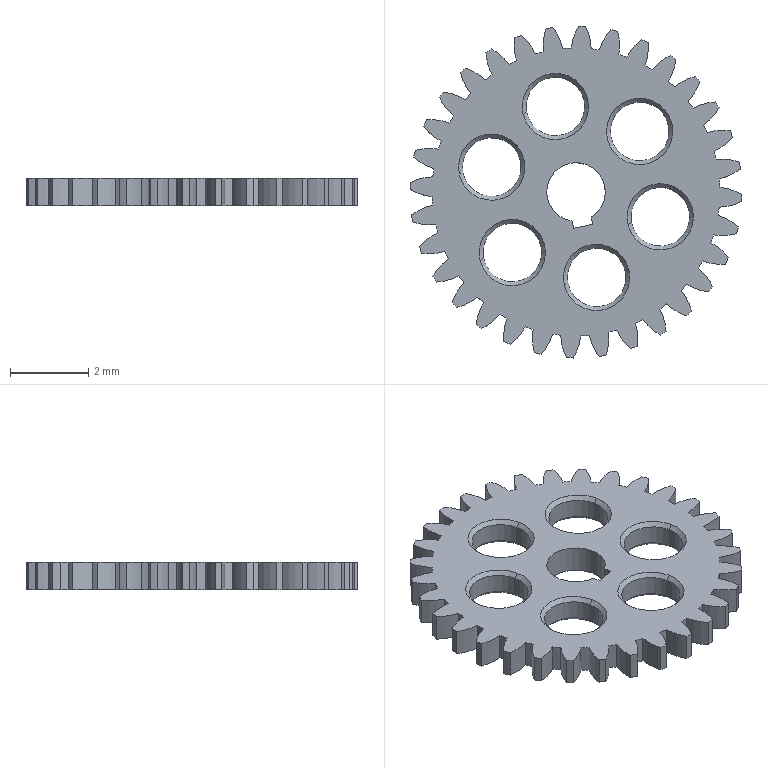Component | SolidWorks | RearServoGear-2 | 1 solid | 176 faces | box 8.5 x 8.5 x 0.7 mm | volume 26 mm3 | cylinder 147 | cone 24 | plane 5 | commonest cylinder face diameters 2.736 x68 7.375 x32 8.5 x32 1.5 x15
build123d program:
from build123d import *

# Parameters (mm, degrees)
SKETCH1_R           = 3.688
SKETCH1_R_2         = 0.75
BOSS_EXTRUDE1_DEPTH = 0.7
BOSS_EXTRUDE2_START = -0.7
BOSS_EXTRUDE2_DEPTH = 0.7
CIRPATTERN1_COUNT   = 32
SKETCH3_R           = 0.75
CUT_EXTRUDE1_DEPTH  = 0.7
CHAMFER1_SIZE       = 0.1
SKETCH4_W           = 0.5
SKETCH4_H           = 0.3
CUT_EXTRUDE2_DEPTH  = 10


with BuildPart() as part:
    # Sketch1 → Boss-Extrude1 (new body)
    with BuildSketch(Plane.XY):
        with Locations((5.25, -3.5)):
            Circle(SKETCH1_R)
        with Locations((5.25, -3.5)):
            Circle(SKETCH1_R_2, mode=Mode.SUBTRACT)
    extrude(amount=BOSS_EXTRUDE1_DEPTH)

    # Sketch2 → Boss-Extrude2 (add)
    with BuildSketch(Plane.XY.offset(0.7).offset(BOSS_EXTRUDE2_START)):
        with BuildLine():
            ThreePointArc((5.547, 0.7396), (5.459, 0.7449), (5.37, 0.7483))
            ThreePointArc((5.37, 0.7483), (5.242, 0.4783), (5.176, 0.187))
            ThreePointArc((5.176, 0.187), (5.431, 0.1833), (5.685, 0.162))
            ThreePointArc((5.685, 0.162), (5.648, 0.4584), (5.547, 0.7396))
        make_face()
    boss_extrude2 = extrude(amount=BOSS_EXTRUDE2_DEPTH)

    # CirPattern1: Boss-Extrude2 ×32 about axis
    cirpattern1_axis = Axis((5.25, -3.5, 0), (0, 0, 1))
    for i in range(1, CIRPATTERN1_COUNT):
        add(boss_extrude2.rotate(cirpattern1_axis, i * 360 / CIRPATTERN1_COUNT))

    # Sketch3 → Cut-Extrude1 (cut)
    with BuildSketch(Plane.XY.offset(0.7)):
        with Locations((3.271, -2.429)):
            Circle(SKETCH3_R)
        with Locations((5.188, -1.251)):
            Circle(SKETCH3_R)
        with Locations((7.167, -2.322)):
            Circle(SKETCH3_R)
        with Locations((7.229, -4.571)):
            Circle(SKETCH3_R)
        with Locations((5.312, -5.749)):
            Circle(SKETCH3_R)
        with Locations((3.333, -4.678)):
            Circle(SKETCH3_R)
    extrude(amount=-CUT_EXTRUDE1_DEPTH, mode=Mode.SUBTRACT)

    # Chamfer1
    chamfer1_edges = [part.edges().sort_by_distance(p)[0] for p in [
        (2.583, -4.678, 0),
        (2.583, -4.678, 0.7),
        (4.562, -5.749, 0),
        (4.562, -5.749, 0.7),
        (6.479, -4.571, 0),
        (6.479, -4.571, 0.7),
        (6.417, -2.322, 0),
        (6.417, -2.322, 0.7),
        (4.438, -1.251, 0),
        (4.438, -1.251, 0.7),
        (2.521, -2.429, 0),
        (2.521, -2.429, 0.7),
    ]]
    chamfer(chamfer1_edges, length=CHAMFER1_SIZE)

    # Sketch4 → Cut-Extrude2 (cut)
    with BuildSketch(Plane.XY):
        with Locations((5.25, -2.75)):
            Rectangle(SKETCH4_W, SKETCH4_H)
    extrude(amount=CUT_EXTRUDE2_DEPTH, mode=Mode.SUBTRACT)


solid = part.part

# Placed as in the assembly
solid = solid.moved(Location((11.612, -5.834, 4.013), (0, 0, -168.025)))